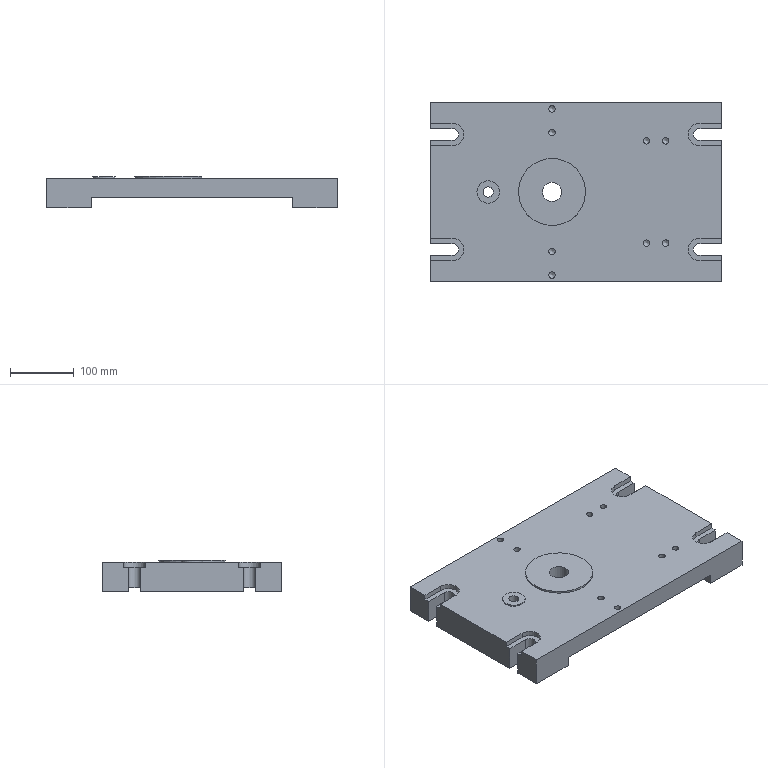Component | NX | FIXTURE_BODY | 1 solid | 80 faces | volume 4253576 mm3 | plane 44 | cylinder 24 | cone 12 | commonest cylinder face diameters 10 x8 18 x4 34 x4 6 x4 105 x1 30 x1 35 x1 16 x1